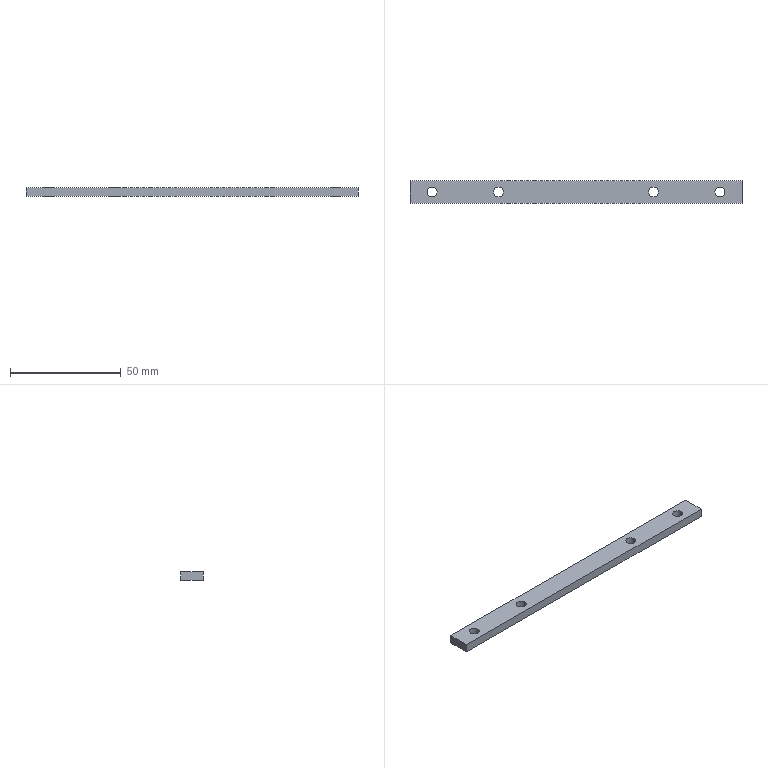CAM job | Mastercam | mm | 8 operations | part box 150 x 10 x 4
1. Facing | 20 - 63 平铣刀
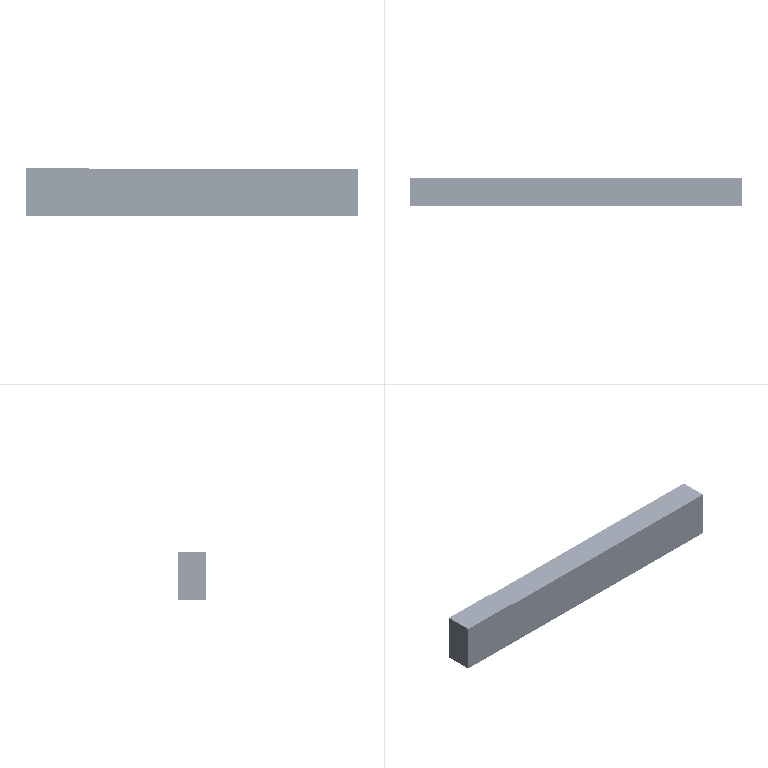2. Contour (Ramp) | 9 - 10 平铣刀
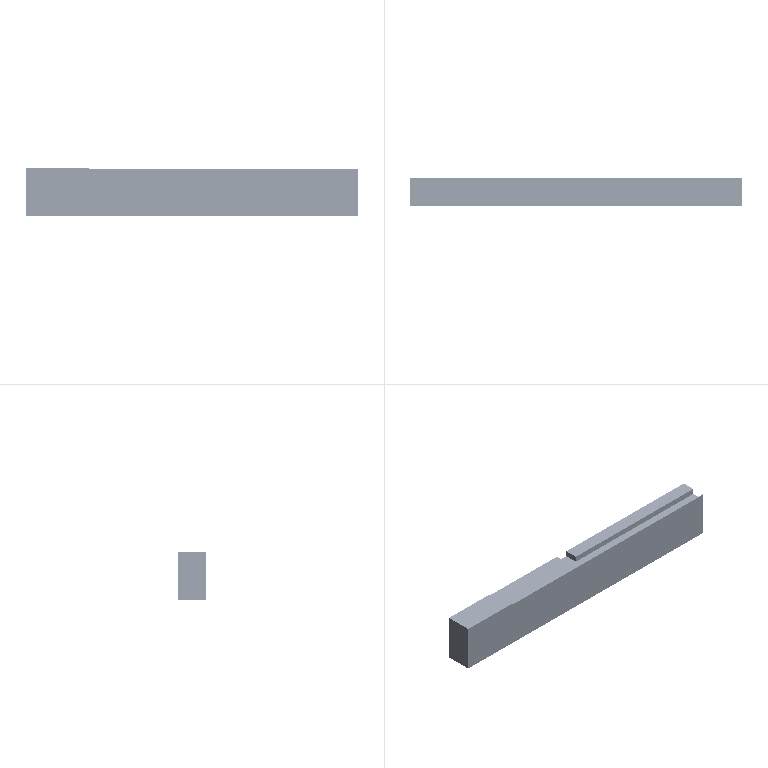3. Contour (2D) | 10 - 10 平铣刀
4. Drill/Counterbore | 7 - 4 倒角刀
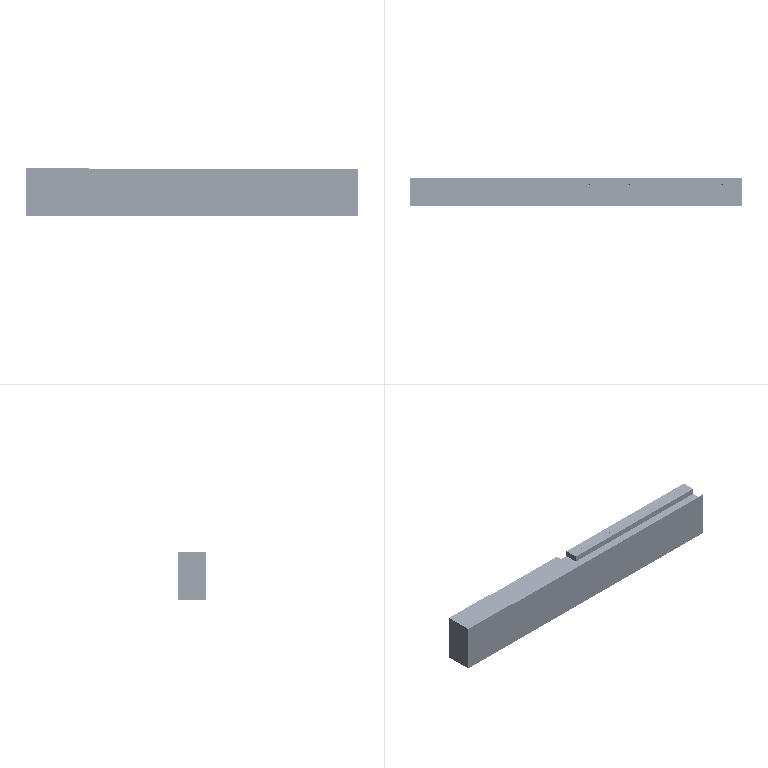5. Contour (2D chamfer) | 7 - 4 倒角刀
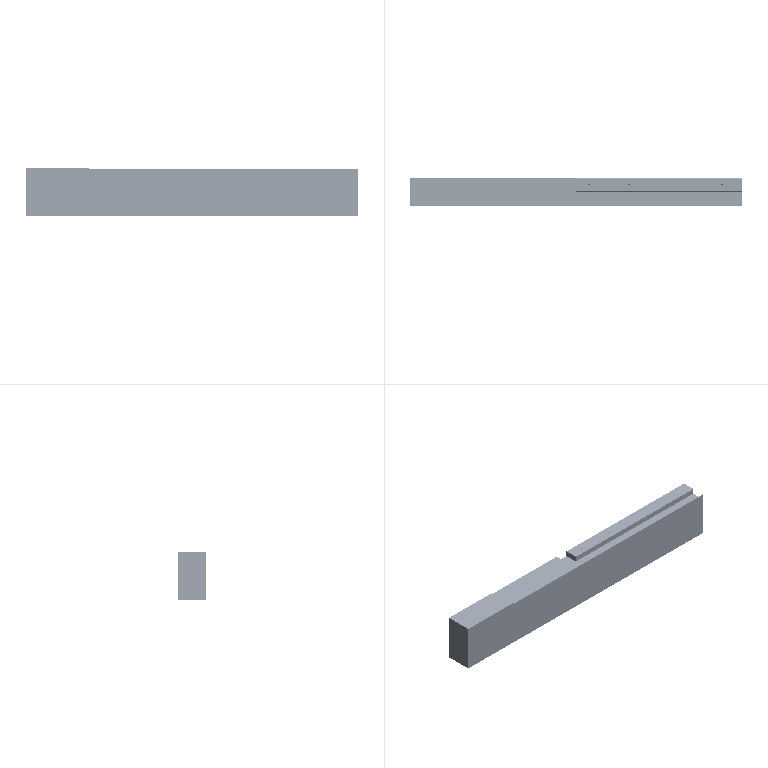6. Facing | 9 - 10 平铣刀
7. Facing | 10 - 10 平铣刀
8. Contour (2D chamfer) | 7 - 4 倒角刀